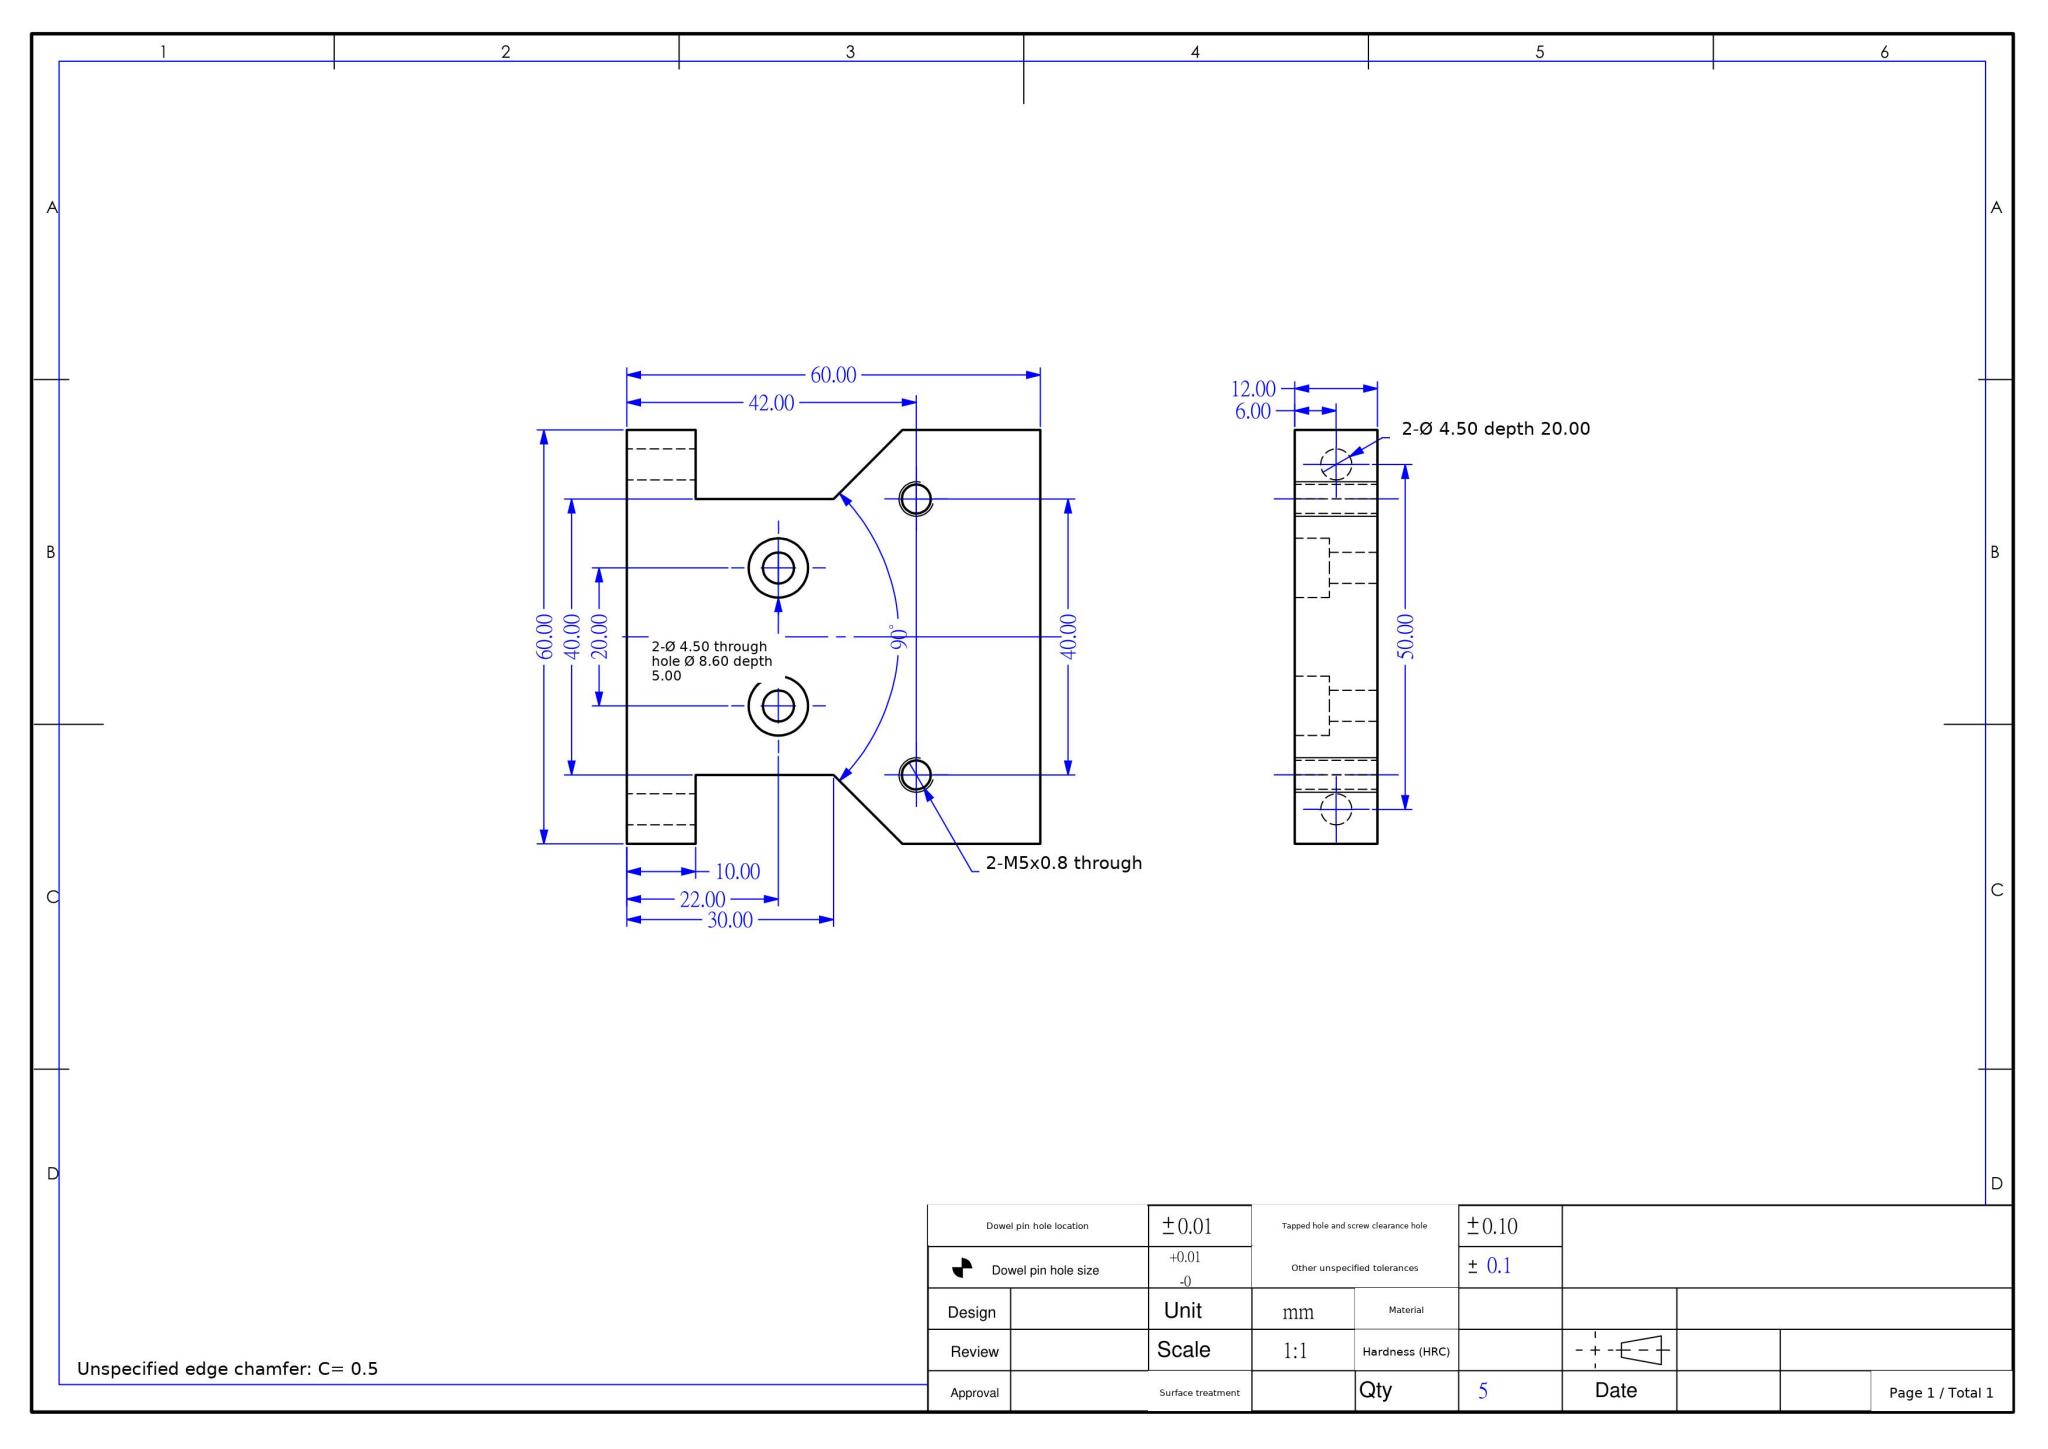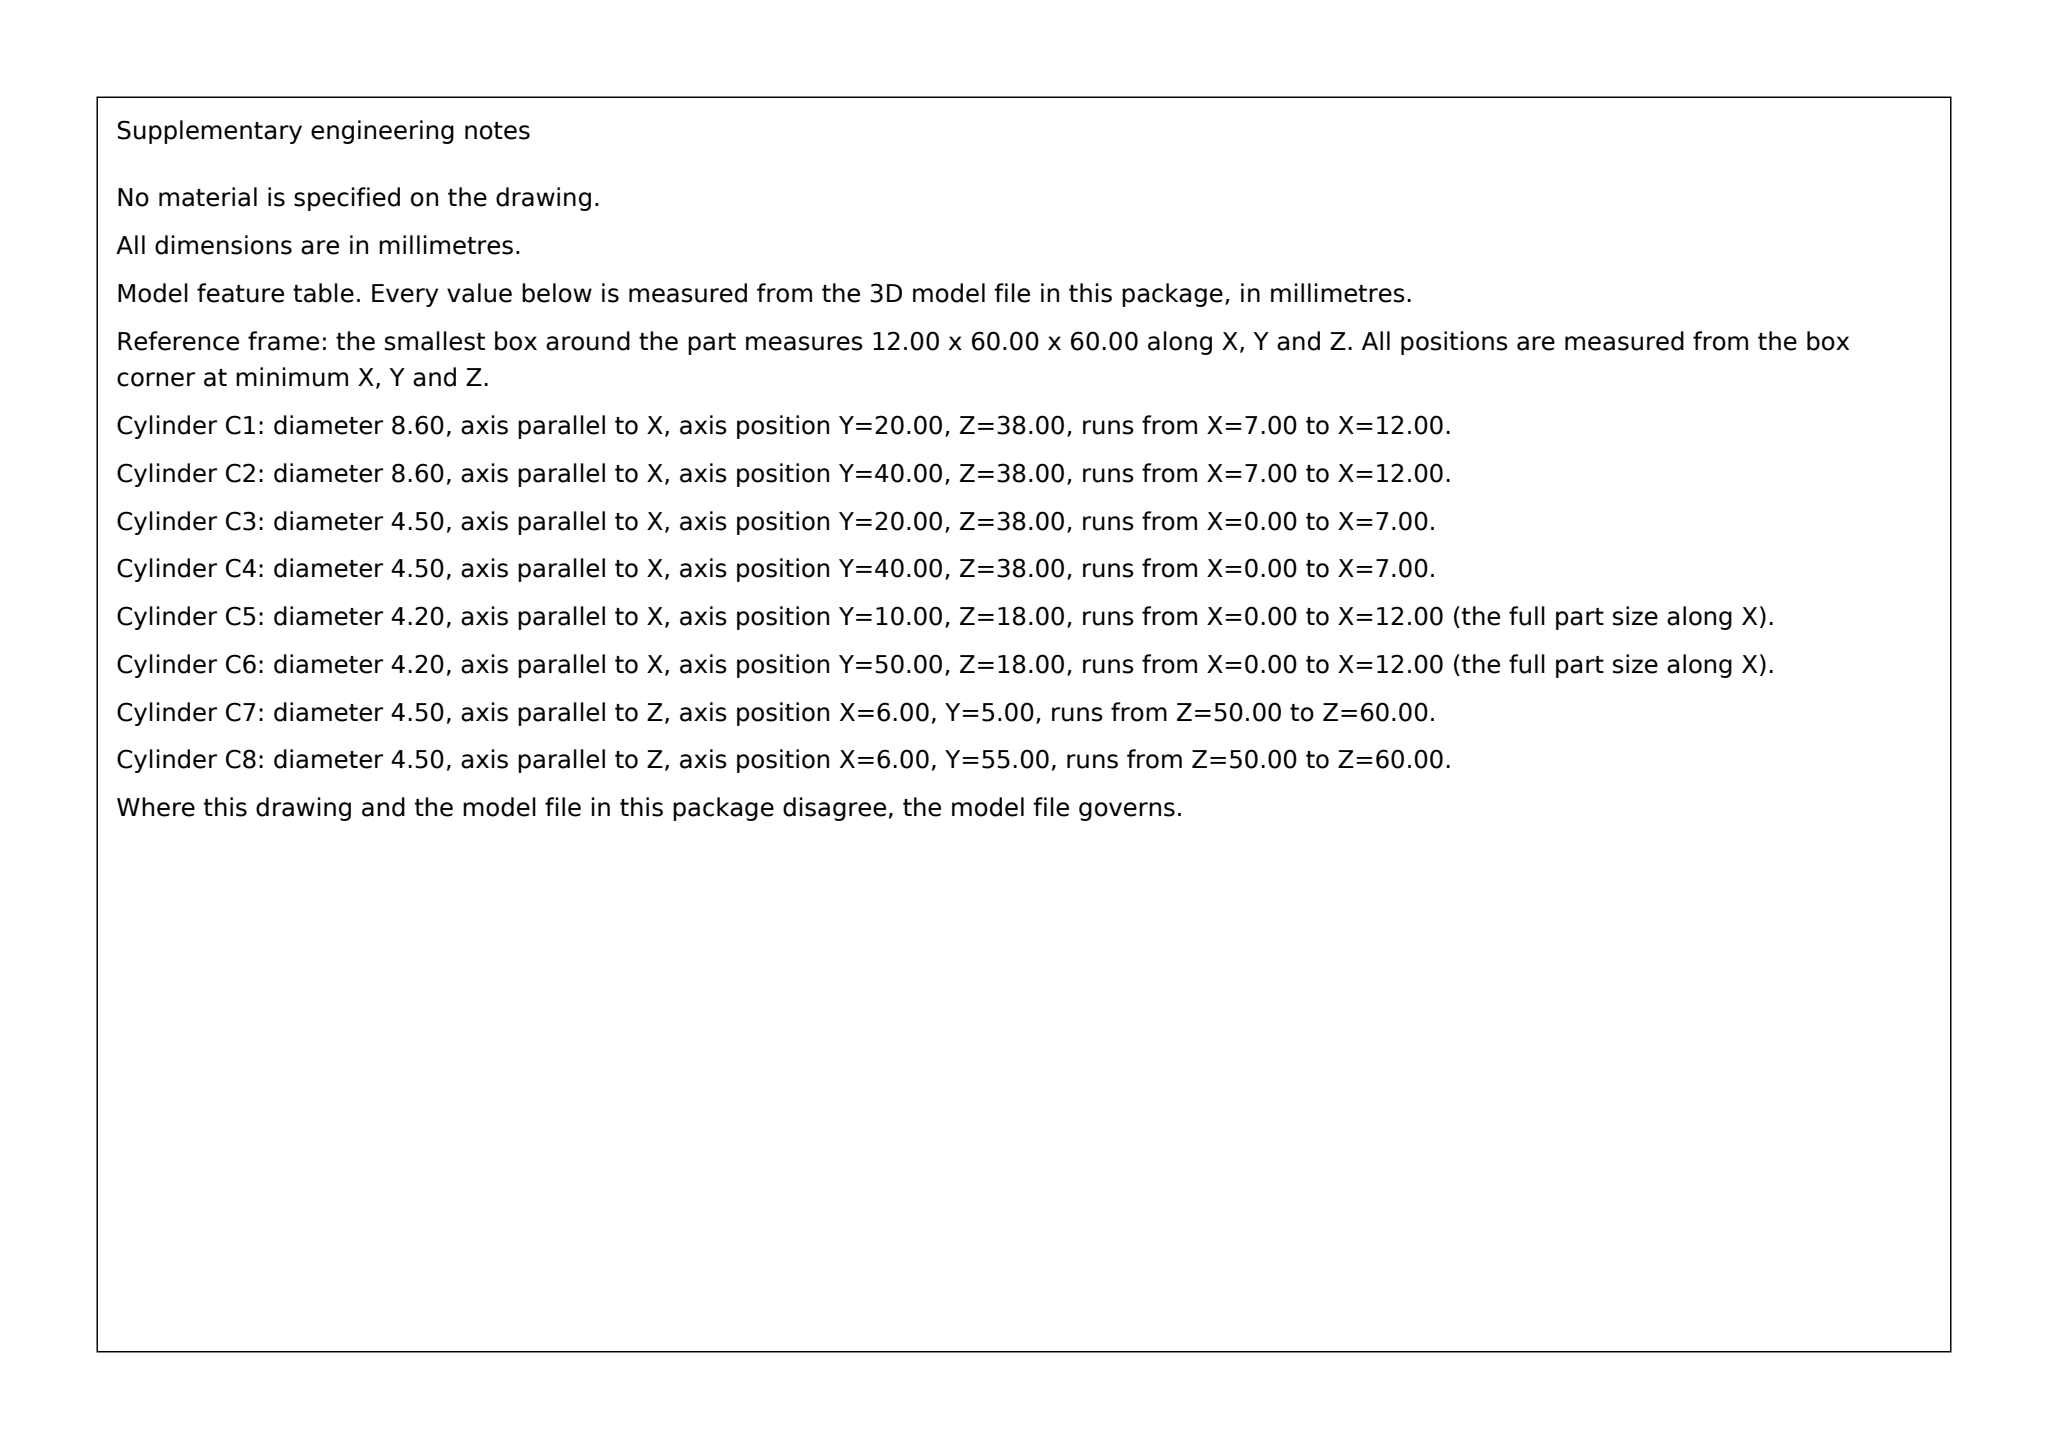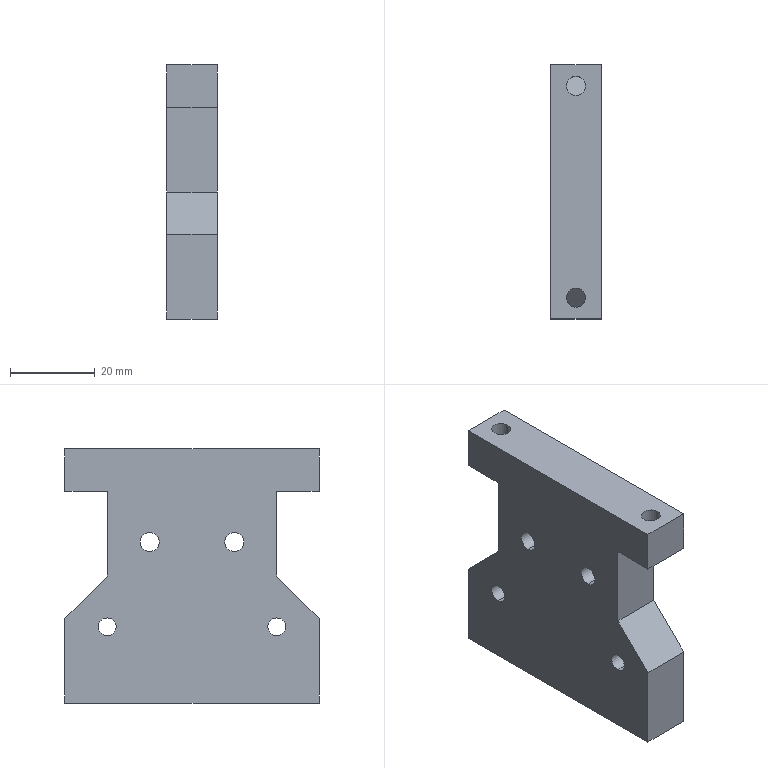Part | SolidWorks | mm | material Plain Carbon Steel | 1 solid | 32 faces | box 12 x 60 x 60 mm | volume 35746 mm3 | cylinder 16 | plane 16 | commonest cylinder face diameters 4.5 x8 8.6 x4 4.2 x4